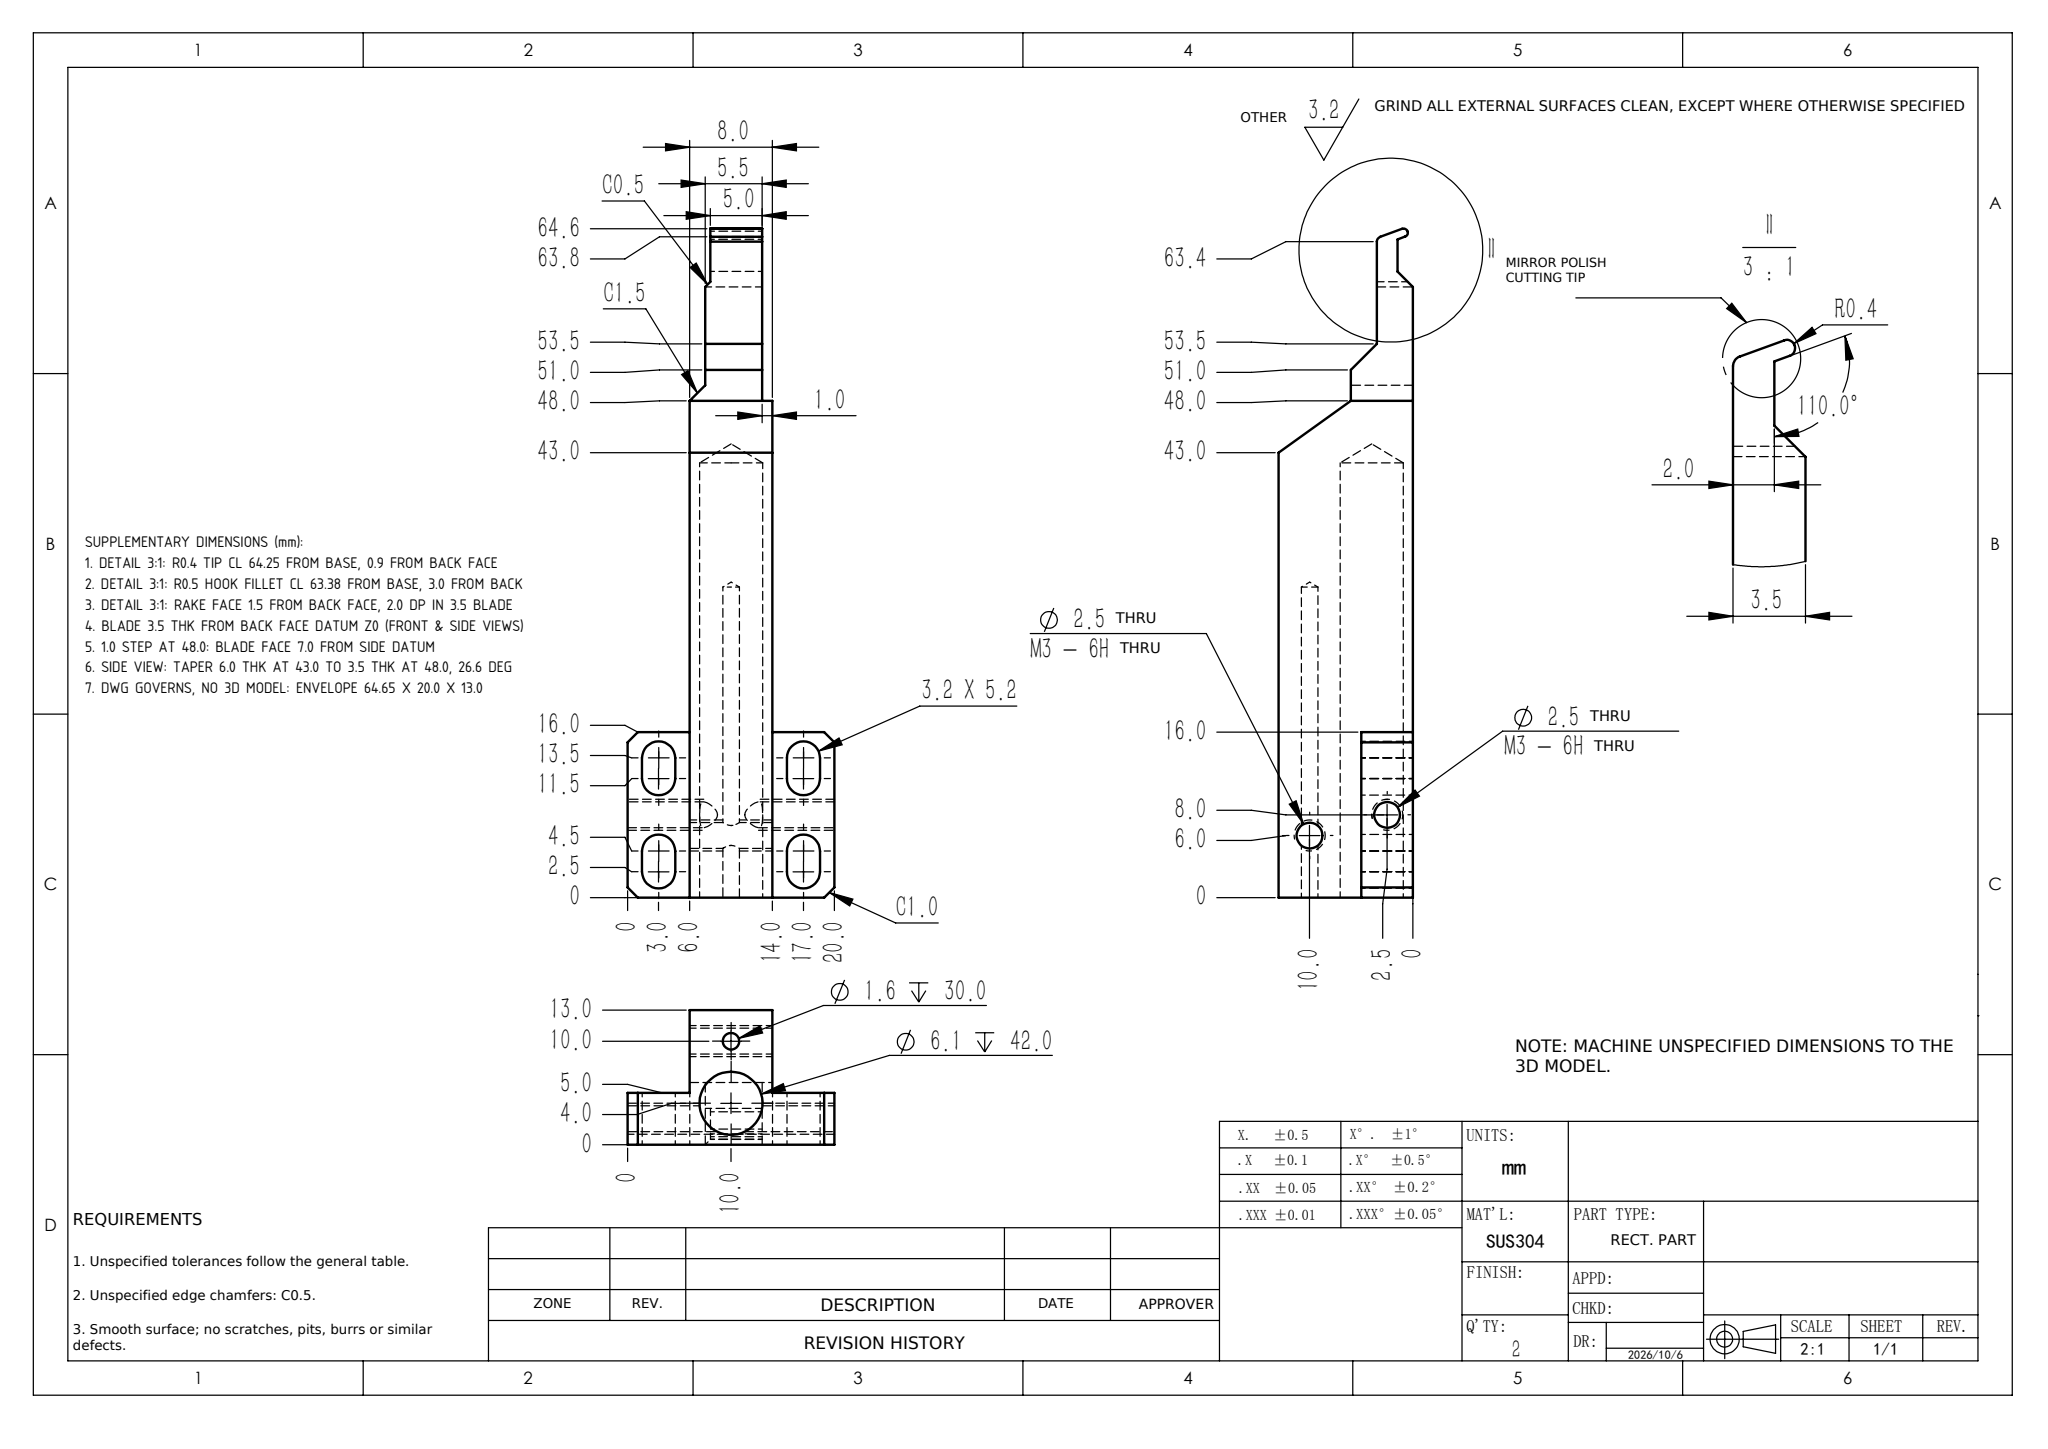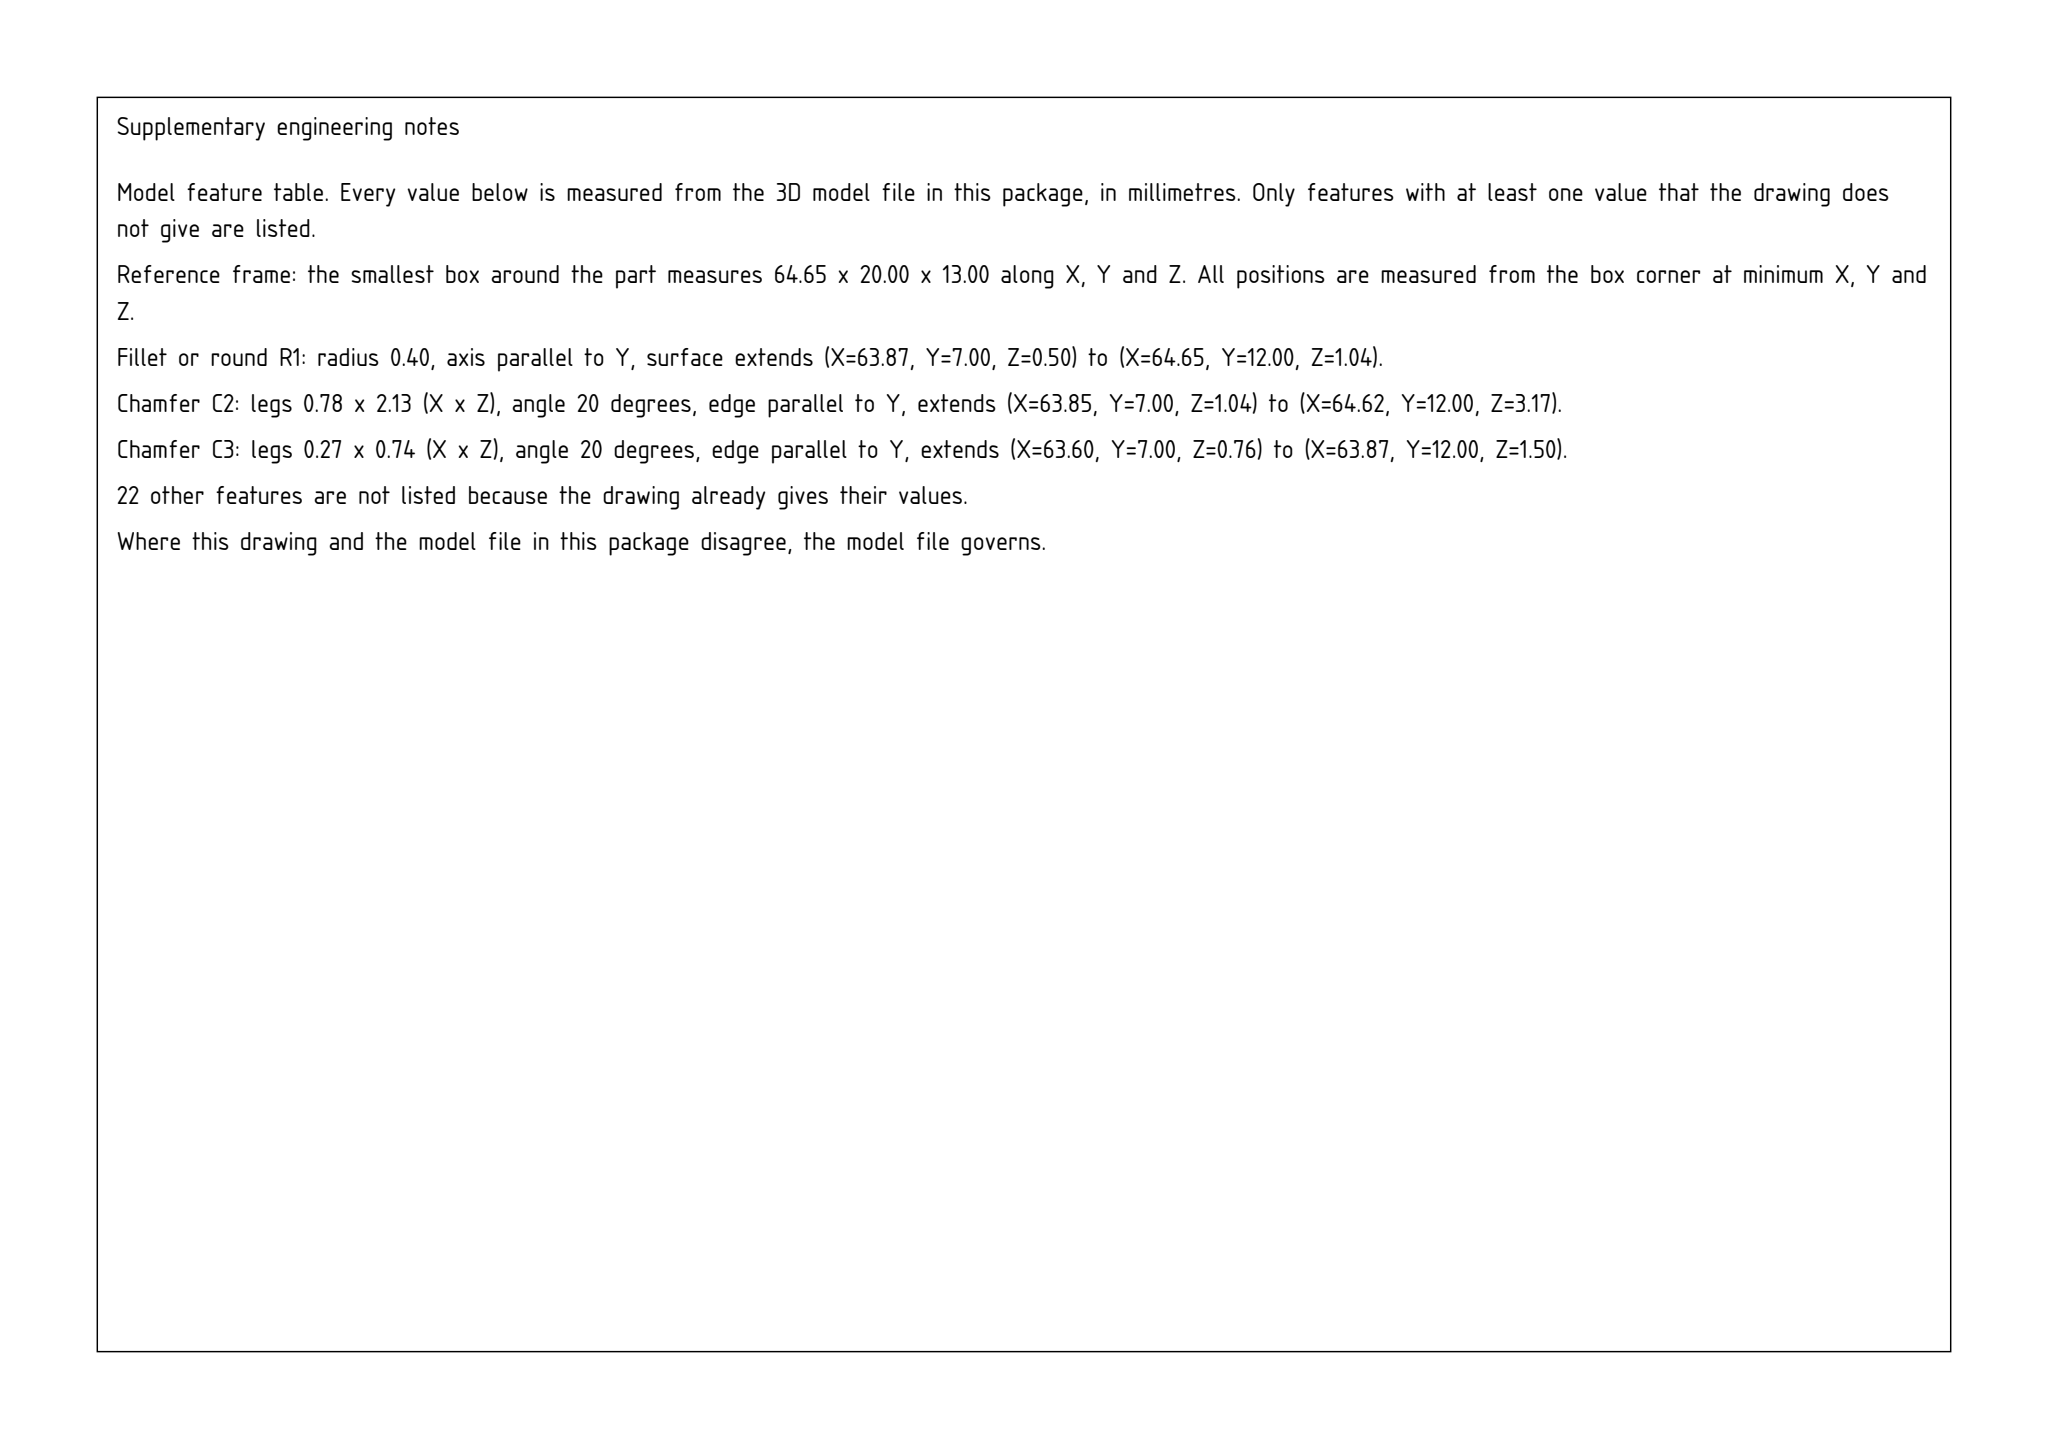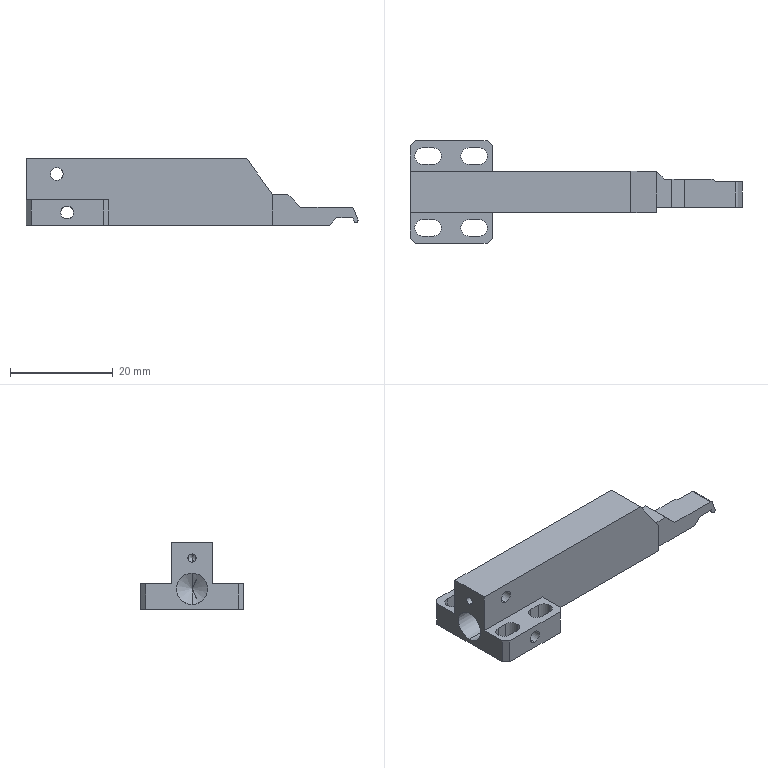Part | SolidWorks | mm | 1 solid | 69 faces | box 64.65 x 20 x 13 mm | volume 4437 mm3 | plane 37 | cylinder 28 | cone 4 | commonest cylinder face diameters 3.2 x12 2.5 x6 1.6 x4 0.8 x3 6.1 x2 1 x1